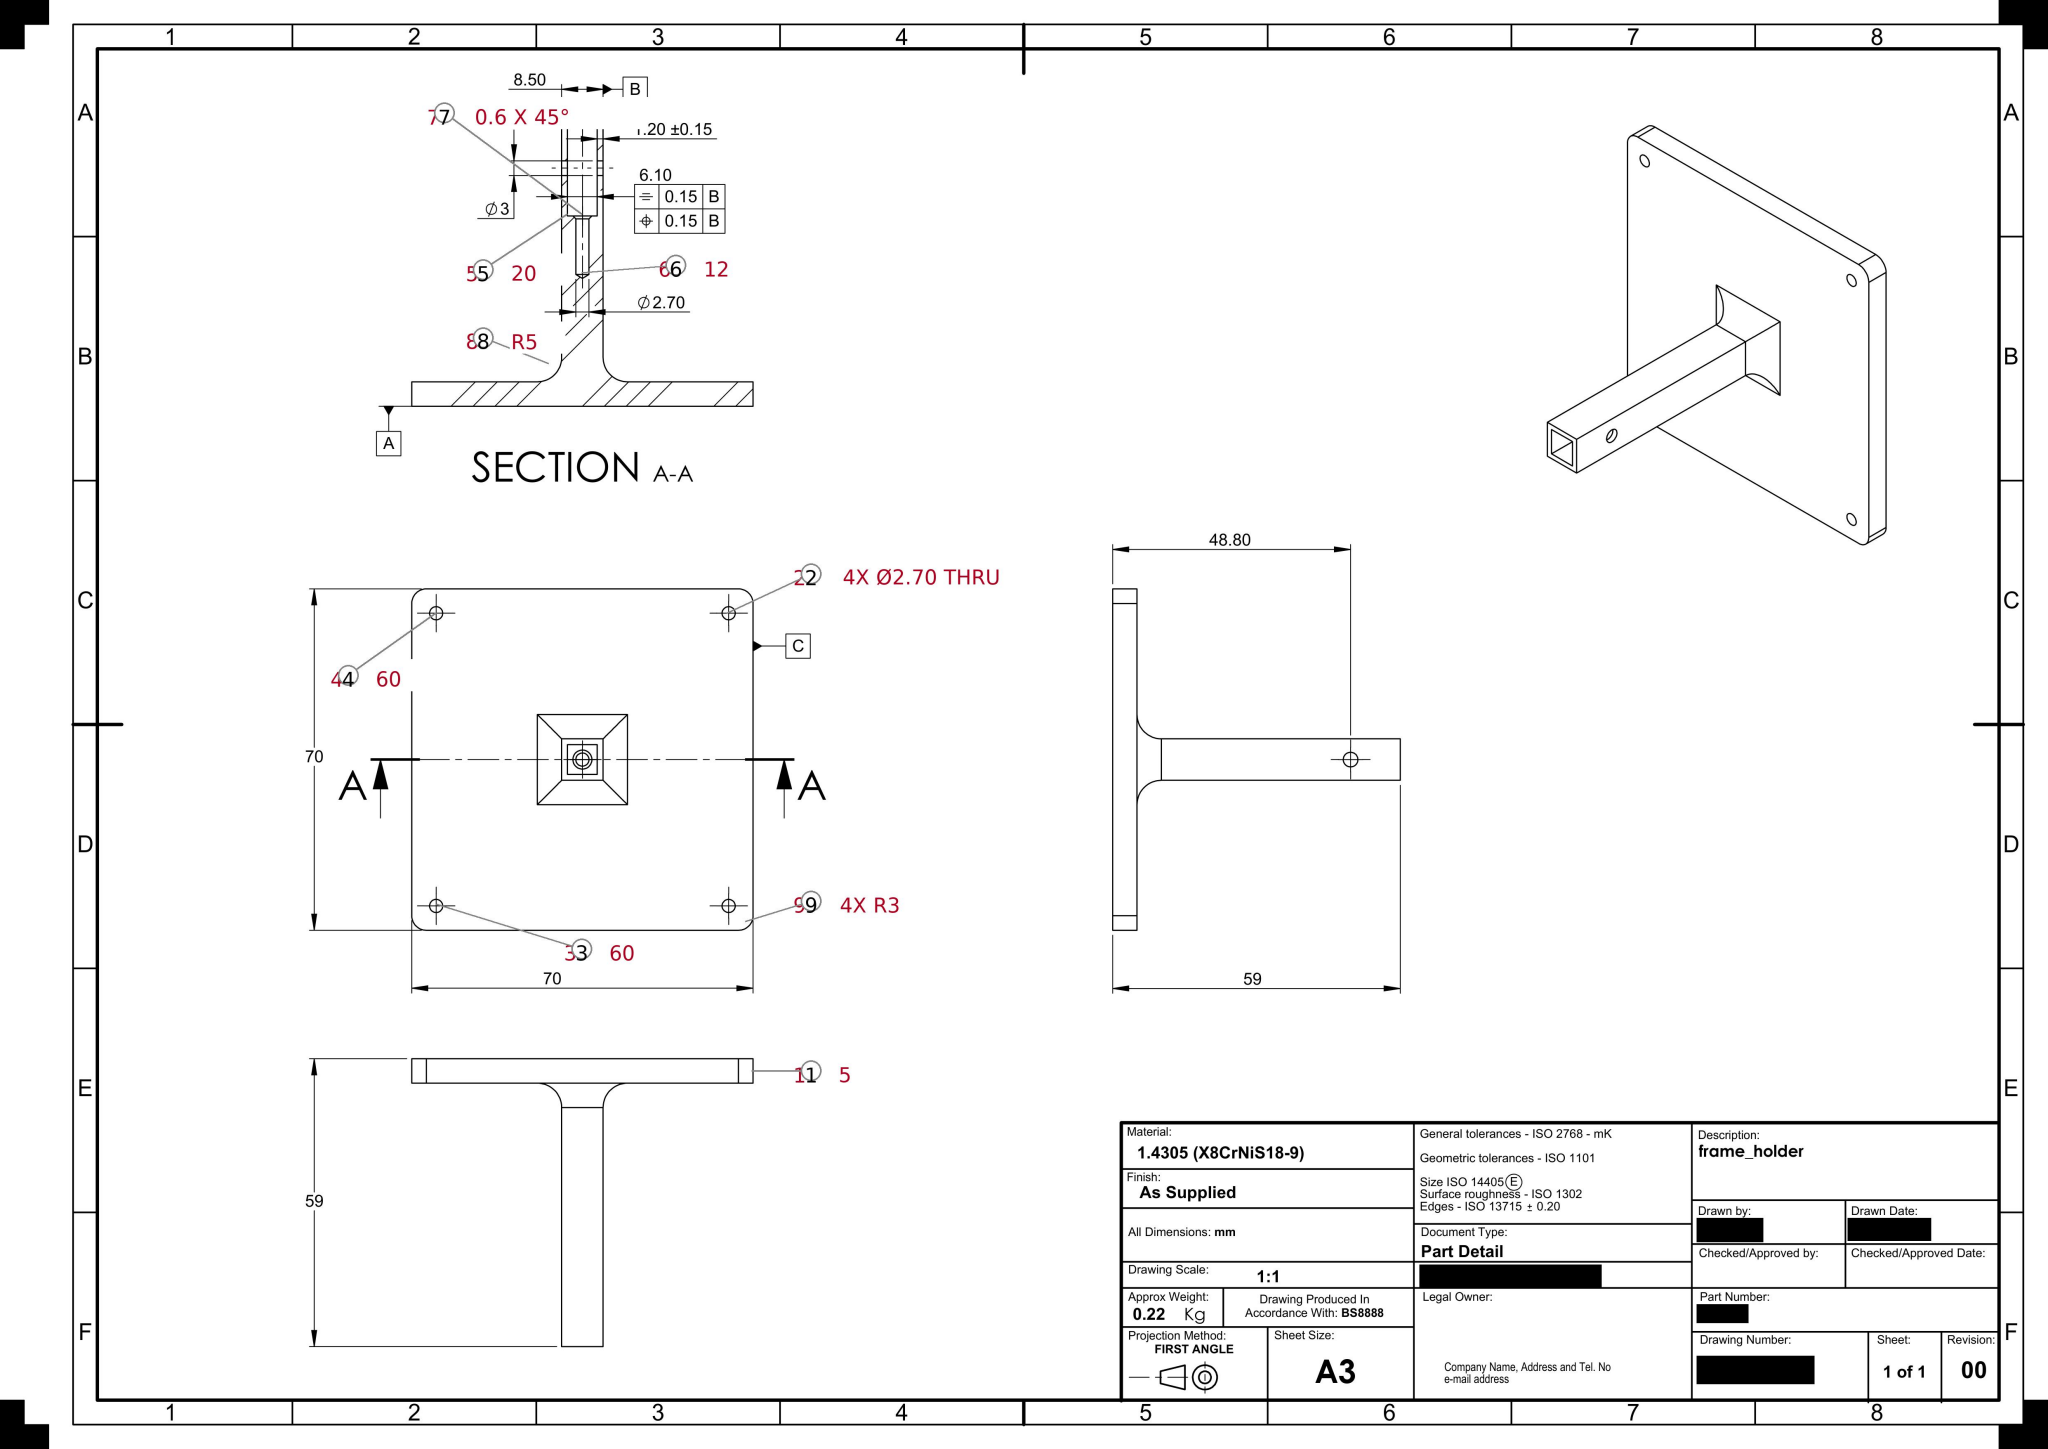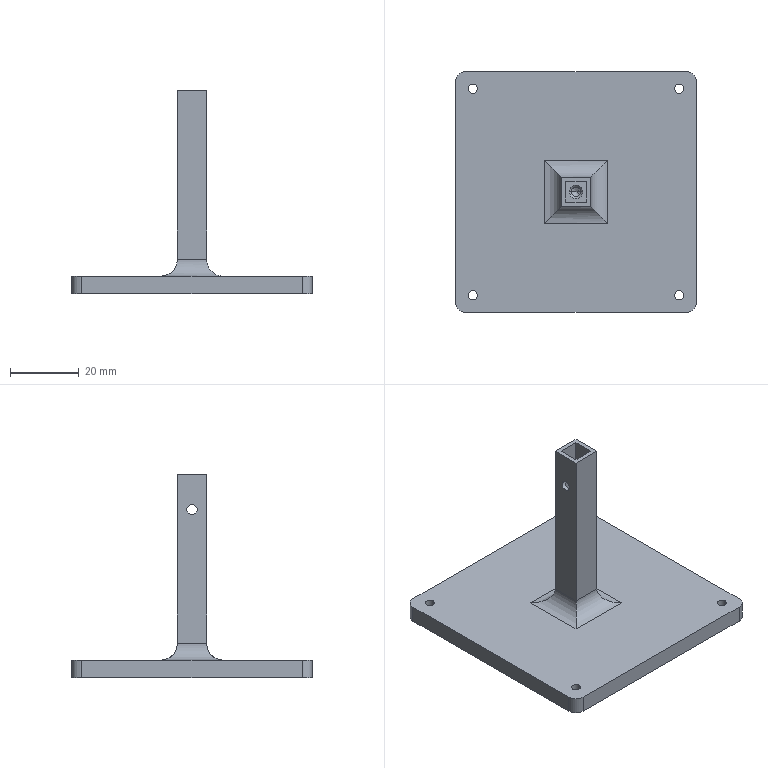Part | SolidWorks | mm | 1 solid | 42 faces | box 70 x 70 x 59 mm | volume 27646 mm3 | cylinder 22 | plane 16 | cone 4 | commonest cylinder face diameters 2.7 x10 3 x4 6 x4 10 x4
build123d program:
from build123d import *

# Parameters (mm, degrees)
SKETCH1_W                            = 70
SKETCH1_H                            = 70
BOSS_EXTRUDE1_DEPTH                  = 5
FILLET1_R                            = 3
SKETCH2_W                            = 8.5
SKETCH2_H                            = 8.5
BOSS_EXTRUDE2_DEPTH                  = 54
FILLET2_R                            = 5
SKETCH3_W                            = 6.1
SKETCH3_H                            = 6.1
CUT_EXTRUDE1_DEPTH                   = 20
SKETCH4_R                            = 1.5
CUT_EXTRUDE2_DEPTH                   = 20
F_2_7_2_7_DIAMETER_HOLE1_D           = 2.7
F_2_7_2_7_DIAMETER_HOLE1_DEPTH       = 12
F_2_7_2_7_DIAMETER_HOLE1_CSINK_D     = 3.9
F_2_7_2_7_DIAMETER_HOLE1_CSINK_ANGLE = 90
F_2_7_2_7_DIAMETER_HOLE1_TIP         = 0.8112
SKETCH8_R                            = 1.35
CUT_EXTRUDE3_DEPTH                   = 20


with BuildPart() as part:
    # Sketch1 → Boss-Extrude1 (new body)
    with BuildSketch(Plane.XY):
        Rectangle(SKETCH1_W, SKETCH1_H)
    extrude(amount=BOSS_EXTRUDE1_DEPTH)

    # Fillet1
    fillet1_edges = [part.edges().sort_by_distance(p)[0] for p in [
        (35, -35, 2.5),
        (-35, -35, 2.5),
        (-35, 35, 2.5),
        (35, 35, 2.5),
    ]]
    fillet(fillet1_edges, radius=FILLET1_R)

    # Sketch2 → Boss-Extrude2 (add)
    with BuildSketch(Plane.XY.offset(5)):
        Rectangle(SKETCH2_W, SKETCH2_H)
    extrude(amount=BOSS_EXTRUDE2_DEPTH)

    # Fillet2
    fillet2_edges = [part.edges().sort_by_distance(p)[0] for p in [
        (4.25, 0, 5),
        (0, 4.25, 5),
        (-4.25, 0, 5),
        (0, -4.25, 5),
    ]]
    fillet(fillet2_edges, radius=FILLET2_R)

    # Sketch3 → Cut-Extrude1 (cut)
    with BuildSketch(Plane.XY.offset(59)):
        Rectangle(SKETCH3_W, SKETCH3_H)
    extrude(amount=-CUT_EXTRUDE1_DEPTH, mode=Mode.SUBTRACT)

    # Sketch4 → Cut-Extrude2 (cut)
    with BuildSketch(Plane(origin=(4.25, 0, 0), x_dir=(0, 0, -1), z_dir=(1, 0, 0))):
        with Locations(Location((-48.8, 0, 0), (0, 0, 90))):
            Circle(SKETCH4_R)
    extrude(amount=-CUT_EXTRUDE2_DEPTH, mode=Mode.SUBTRACT)

    # 2.7 _2.7_ Diameter Hole1
    with Locations(Plane.XY.offset(39)):
        with Locations((0, 0)):
            CounterSinkHole(F_2_7_2_7_DIAMETER_HOLE1_D / 2, F_2_7_2_7_DIAMETER_HOLE1_CSINK_D / 2, depth=F_2_7_2_7_DIAMETER_HOLE1_DEPTH, counter_sink_angle=F_2_7_2_7_DIAMETER_HOLE1_CSINK_ANGLE)
            with Locations((0, 0, -(F_2_7_2_7_DIAMETER_HOLE1_DEPTH + F_2_7_2_7_DIAMETER_HOLE1_TIP / 2))):  # 118° drill point
                Cone(0, F_2_7_2_7_DIAMETER_HOLE1_D / 2, F_2_7_2_7_DIAMETER_HOLE1_TIP, mode=Mode.SUBTRACT)

    # Sketch8 → Cut-Extrude3 (cut)
    with BuildSketch(Plane.XY.offset(5)):
        with Locations((30, -30)):
            Circle(SKETCH8_R)
        with Locations((30, 30)):
            Circle(SKETCH8_R)
        with Locations((-30, 30)):
            Circle(SKETCH8_R)
        with Locations((-30, -30)):
            Circle(SKETCH8_R)
    extrude(amount=-CUT_EXTRUDE3_DEPTH, mode=Mode.SUBTRACT)


solid = part.part